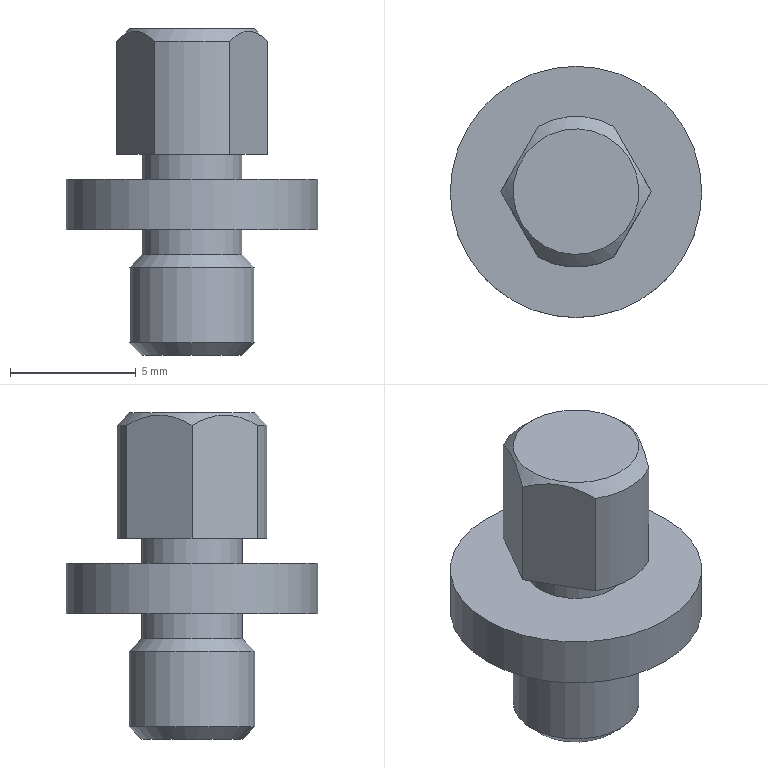Component | NX | DIAMOND_PIN | 1 solid | 18 faces | volume 381 mm3 | plane 9 | cylinder 6 | cone 3 | commonest cylinder face diameters 4 x2 6 x2 5 x1 10 x1